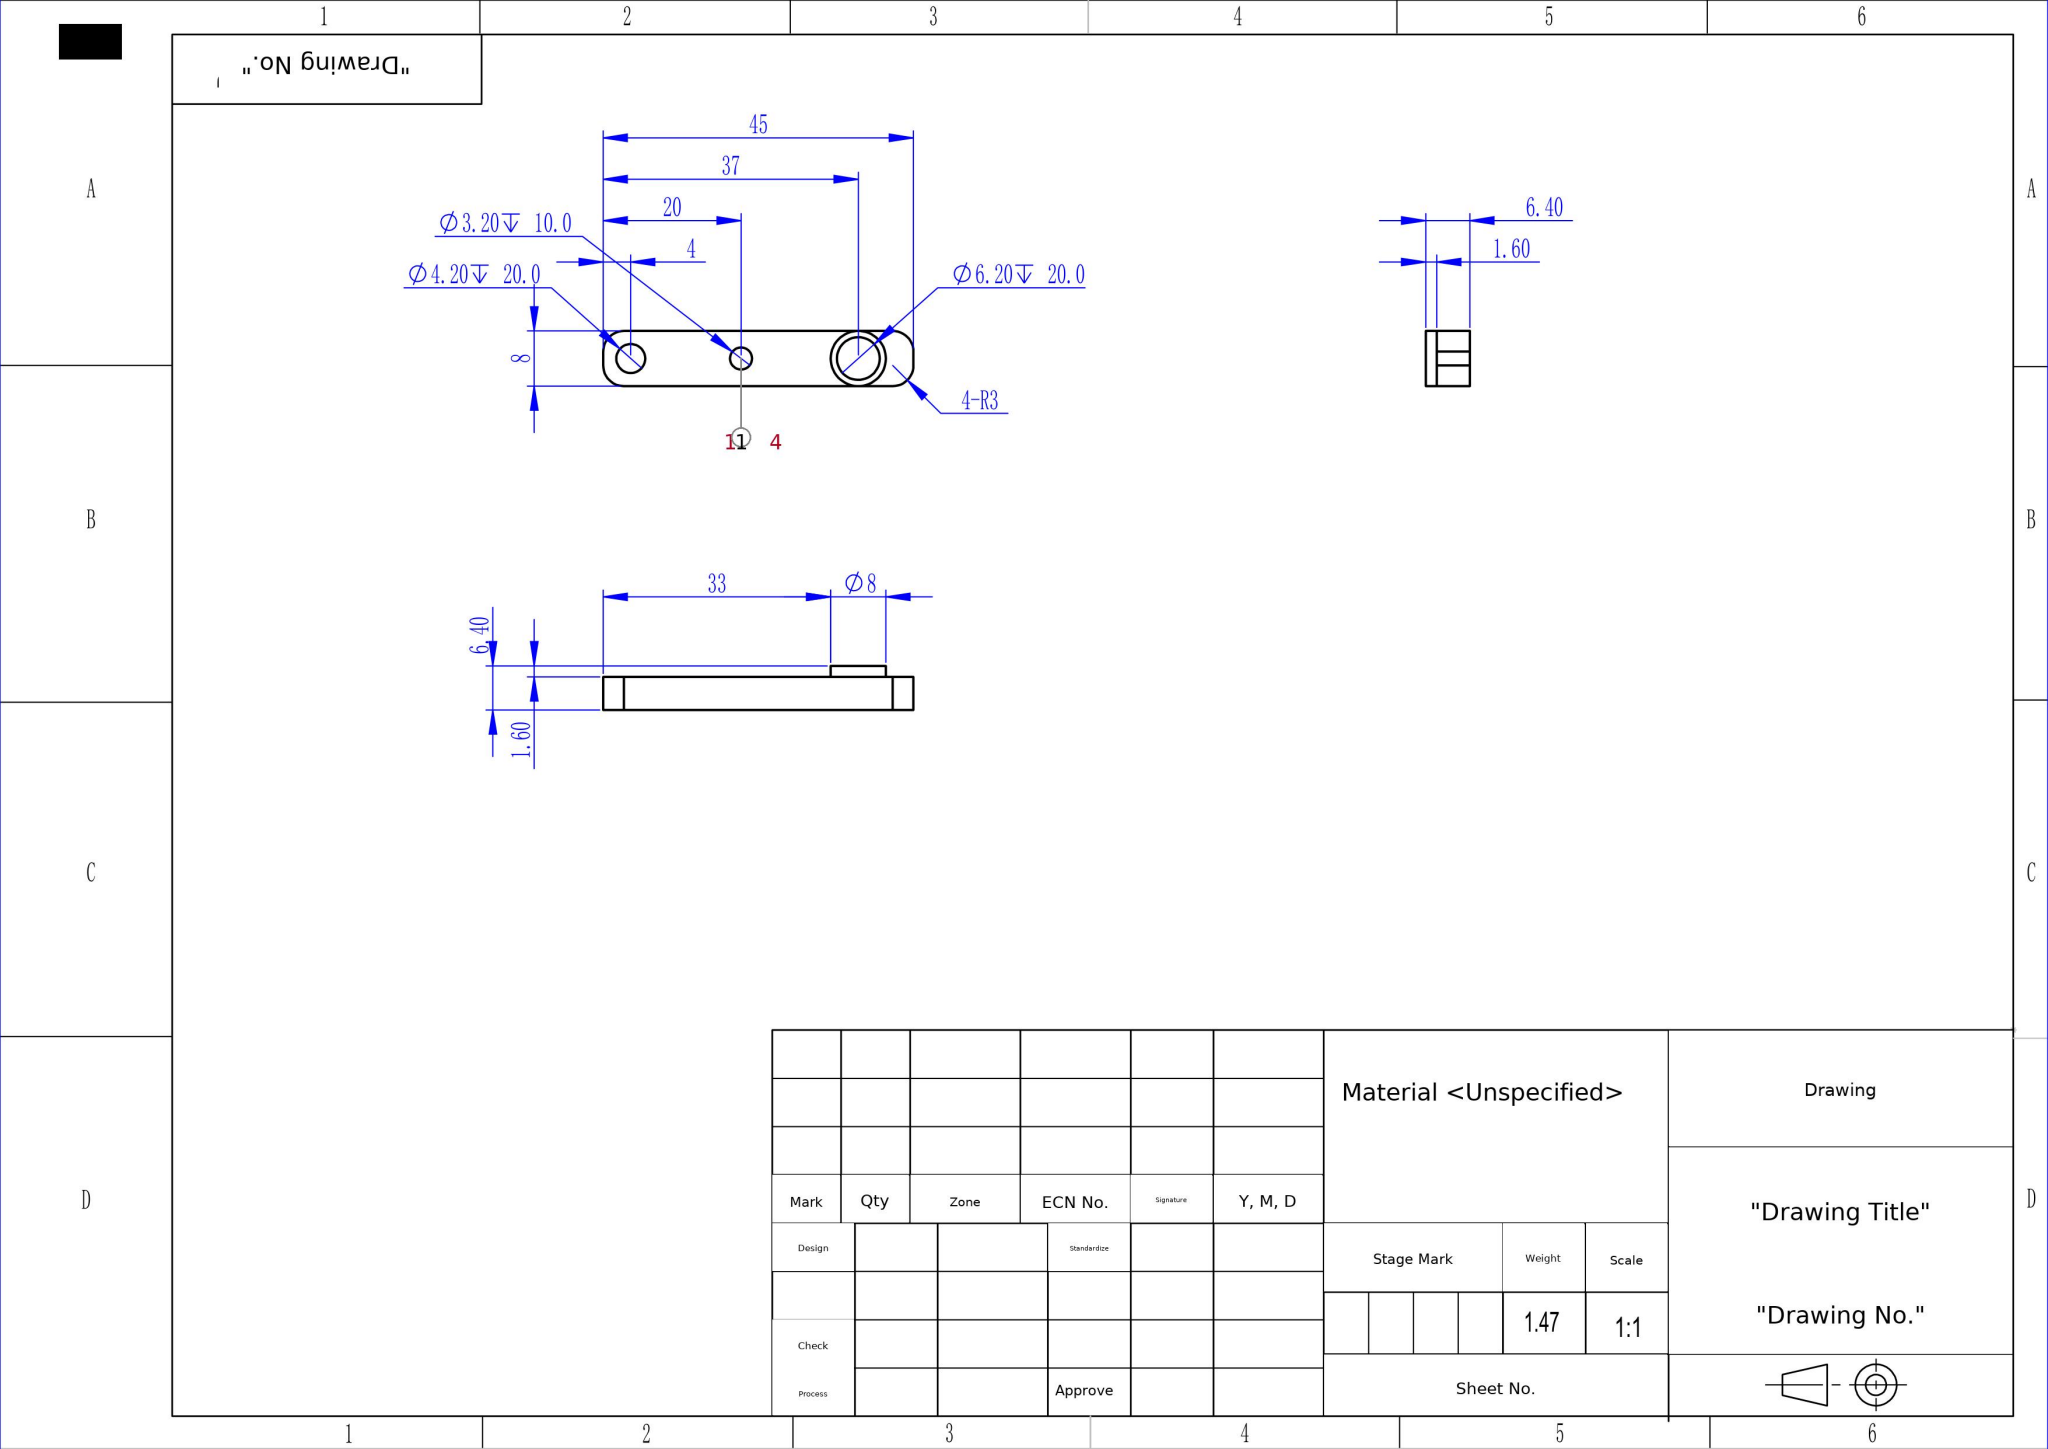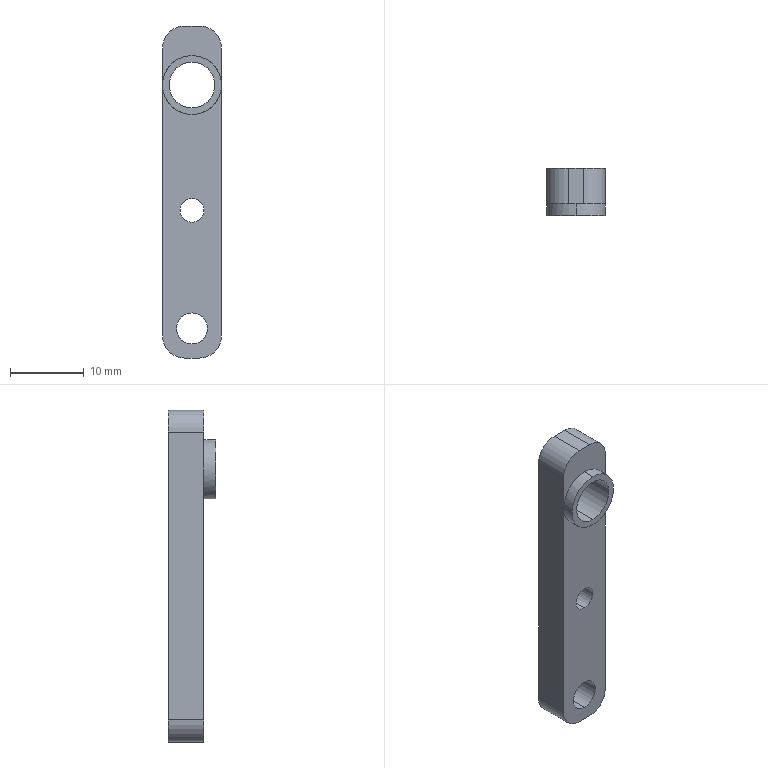Part | SolidWorks | mm | material Unspecified | 1 solid | 20 faces | box 8 x 6.4 x 45 mm | volume 1473 mm3 | cylinder 12 | plane 8 | commonest cylinder face diameters 6 x4 3.2 x2 8 x2 6.2 x2 4.2 x2
build123d program:
from build123d import *

# Parameters (mm, degrees)
SKETCH1_W           = 8
SKETCH1_H           = 4.8
BOSS_EXTRUDE1_DEPTH = 45
SKETCH2_R           = 2.1
CUT_EXTRUDE1_DEPTH  = 20
FILLET1_R           = 3
SKETCH3_R           = 3.1
CUT_EXTRUDE2_DEPTH  = 20
FILLET2_R           = 3
SKETCH4_R           = 4
SKETCH4_R_2         = 3.1
BOSS_EXTRUDE2_DEPTH = 1.6
SKETCH5_R           = 1.6
CUT_EXTRUDE3_DEPTH  = 10


with BuildPart() as part:
    # Sketch1 → Boss-Extrude1 (new body)
    with BuildSketch(Plane.XY):
        Rectangle(SKETCH1_W, SKETCH1_H)
    extrude(amount=BOSS_EXTRUDE1_DEPTH)

    # Sketch2 → Cut-Extrude1 (cut)
    with BuildSketch(Plane(origin=(0, 2.4, 0), x_dir=(1, 0, 0), z_dir=(0, 1, 0))):
        with Locations(Location((0, -4, 0), (0, 0, 270))):
            Circle(SKETCH2_R)
    extrude(amount=-CUT_EXTRUDE1_DEPTH, mode=Mode.SUBTRACT)

    # Fillet1
    fillet1_edges = [part.edges().sort_by_distance(p)[0] for p in [
        (-4, 0, 0),
        (4, 0, 0),
    ]]
    fillet(fillet1_edges, radius=FILLET1_R)

    # Sketch3 → Cut-Extrude2 (cut)
    with BuildSketch(Plane(origin=(0, 2.4, 0), x_dir=(1, 0, 0), z_dir=(0, 1, 0))):
        with Locations(Location((0, -37, 0), (0, 0, 270))):
            Circle(SKETCH3_R)
    extrude(amount=-CUT_EXTRUDE2_DEPTH, mode=Mode.SUBTRACT)

    # Fillet2
    fillet2_edges = [part.edges().sort_by_distance(p)[0] for p in [
        (-4, 0, 45),
        (4, 0, 45),
    ]]
    fillet(fillet2_edges, radius=FILLET2_R)

    # Sketch4 → Boss-Extrude2 (add)
    with BuildSketch(Plane.XZ.offset(2.4)):
        with Locations(Location((0, 37, 0), (0, 0, 90))):
            Circle(SKETCH4_R)
        with Locations(Location((0, 37, 0), (0, 0, 90))):
            Circle(SKETCH4_R_2, mode=Mode.SUBTRACT)
    extrude(amount=BOSS_EXTRUDE2_DEPTH)

    # Sketch5 → Cut-Extrude3 (cut)
    with BuildSketch(Plane(origin=(0, 2.4, 0), x_dir=(1, 0, 0), z_dir=(0, 1, 0))):
        with Locations(Location((0, -20, 0), (0, 0, 270))):
            Circle(SKETCH5_R)
    extrude(amount=-CUT_EXTRUDE3_DEPTH, mode=Mode.SUBTRACT)


solid = part.part
STEP:
#1=CARTESIAN_POINT('',(0.,-2.4,18.4));
#2=VERTEX_POINT('',#1);
#3=CARTESIAN_POINT('',(0.,-2.4,21.6));
#4=VERTEX_POINT('',#3);
#5=CARTESIAN_POINT('',(0.,-2.4,20.));
#6=DIRECTION('',(0.,1.,0.));
#7=DIRECTION('',(0.,0.,1.));
#8=AXIS2_PLACEMENT_3D('',#5,#6,#7);
#9=CIRCLE('',#8,1.6);
#10=EDGE_CURVE('',#2,#4,#9,.T.);
#11=ORIENTED_EDGE('',*,*,#10,.F.);
#12=CARTESIAN_POINT('',(0.,2.4,18.4));
#13=VERTEX_POINT('',#12);
#14=CARTESIAN_POINT('',(0.,-7.6,18.4));
#15=DIRECTION('',(0.,1.,0.));
#16=VECTOR('',#15,1000.);
#17=LINE('',#14,#16);
#18=EDGE_CURVE('',#2,#13,#17,.T.);
#19=ORIENTED_EDGE('',*,*,#18,.T.);
#20=CARTESIAN_POINT('',(0.,2.4,21.6));
#21=VERTEX_POINT('',#20);
#22=CARTESIAN_POINT('',(0.,2.4,20.));
#23=DIRECTION('',(0.,1.,0.));
#24=DIRECTION('',(0.,0.,1.));
#25=AXIS2_PLACEMENT_3D('',#22,#23,#24);
#26=CIRCLE('',#25,1.6);
#27=EDGE_CURVE('',#13,#21,#26,.T.);
#28=ORIENTED_EDGE('',*,*,#27,.T.);
#29=CARTESIAN_POINT('',(0.,-7.6,21.6));
#30=DIRECTION('',(0.,1.,0.));
#31=VECTOR('',#30,1000.);
#32=LINE('',#29,#31);
#33=EDGE_CURVE('',#4,#21,#32,.T.);
#34=ORIENTED_EDGE('',*,*,#33,.F.);
#35=EDGE_LOOP('',(#11,#19,#28,#34));
#36=FACE_OUTER_BOUND('',#35,.T.);
#37=CARTESIAN_POINT('',(0.,-7.6,20.));
#38=DIRECTION('',(0.,1.,0.));
#39=DIRECTION('',(0.,0.,1.));
#40=AXIS2_PLACEMENT_3D('',#37,#38,#39);
#41=CYLINDRICAL_SURFACE('',#40,1.6);
#42=ADVANCED_FACE('',(#36),#41,.F.);
#43=CARTESIAN_POINT('',(0.,-4.,41.));
#44=VERTEX_POINT('',#43);
#45=CARTESIAN_POINT('',(0.,-4.,33.));
#46=VERTEX_POINT('',#45);
#47=CARTESIAN_POINT('',(0.,-4.,37.));
#48=DIRECTION('',(0.,1.,-0.));
#49=DIRECTION('',(0.,0.,1.));
#50=AXIS2_PLACEMENT_3D('',#47,#48,#49);
#51=CIRCLE('',#50,4.);
#52=EDGE_CURVE('',#44,#46,#51,.T.);
#53=ORIENTED_EDGE('',*,*,#52,.T.);
#54=CARTESIAN_POINT('',(0.,-2.4,33.));
#55=VERTEX_POINT('',#54);
#56=CARTESIAN_POINT('',(0.,-15.314,33.));
#57=DIRECTION('',(0.,1.,0.));
#58=VECTOR('',#57,1000.);
#59=LINE('',#56,#58);
#60=EDGE_CURVE('',#46,#55,#59,.T.);
#61=ORIENTED_EDGE('',*,*,#60,.T.);
#62=CARTESIAN_POINT('',(4.,-2.4,37.));
#63=VERTEX_POINT('',#62);
#64=CARTESIAN_POINT('',(0.,-2.4,37.));
#65=DIRECTION('',(0.,-1.,0.));
#66=DIRECTION('',(0.,0.,-1.));
#67=AXIS2_PLACEMENT_3D('',#64,#65,#66);
#68=CIRCLE('',#67,4.);
#69=EDGE_CURVE('',#55,#63,#68,.T.);
#70=ORIENTED_EDGE('',*,*,#69,.T.);
#71=CARTESIAN_POINT('',(0.,-2.4,41.));
#72=VERTEX_POINT('',#71);
#73=CARTESIAN_POINT('',(0.,-2.4,37.));
#74=DIRECTION('',(0.,-1.,0.));
#75=DIRECTION('',(0.,0.,-1.));
#76=AXIS2_PLACEMENT_3D('',#73,#74,#75);
#77=CIRCLE('',#76,4.);
#78=EDGE_CURVE('',#63,#72,#77,.T.);
#79=ORIENTED_EDGE('',*,*,#78,.T.);
#80=CARTESIAN_POINT('',(0.,-15.314,41.));
#81=DIRECTION('',(0.,1.,0.));
#82=VECTOR('',#81,1000.);
#83=LINE('',#80,#82);
#84=EDGE_CURVE('',#44,#72,#83,.T.);
#85=ORIENTED_EDGE('',*,*,#84,.F.);
#86=EDGE_LOOP('',(#53,#61,#70,#79,#85));
#87=FACE_OUTER_BOUND('',#86,.T.);
#88=CARTESIAN_POINT('',(0.,-15.314,37.));
#89=DIRECTION('',(0.,1.,0.));
#90=DIRECTION('',(0.,0.,1.));
#91=AXIS2_PLACEMENT_3D('',#88,#89,#90);
#92=CYLINDRICAL_SURFACE('',#91,4.);
#93=ADVANCED_FACE('',(#87),#92,.T.);
#94=CARTESIAN_POINT('',(0.,-4.,33.9));
#95=VERTEX_POINT('',#94);
#96=CARTESIAN_POINT('',(0.,-4.,40.1));
#97=VERTEX_POINT('',#96);
#98=CARTESIAN_POINT('',(0.,-4.,37.));
#99=DIRECTION('',(0.,1.,-0.));
#100=DIRECTION('',(0.,0.,1.));
#101=AXIS2_PLACEMENT_3D('',#98,#99,#100);
#102=CIRCLE('',#101,3.1);
#103=EDGE_CURVE('',#95,#97,#102,.T.);
#104=ORIENTED_EDGE('',*,*,#103,.F.);
#105=CARTESIAN_POINT('',(0.,2.4,33.9));
#106=VERTEX_POINT('',#105);
#107=CARTESIAN_POINT('',(0.,-17.6,33.9));
#108=DIRECTION('',(0.,1.,0.));
#109=VECTOR('',#108,1000.);
#110=LINE('',#107,#109);
#111=EDGE_CURVE('',#95,#106,#110,.T.);
#112=ORIENTED_EDGE('',*,*,#111,.T.);
#113=CARTESIAN_POINT('',(0.,2.4,40.1));
#114=VERTEX_POINT('',#113);
#115=CARTESIAN_POINT('',(0.,2.4,37.));
#116=DIRECTION('',(0.,1.,0.));
#117=DIRECTION('',(0.,0.,1.));
#118=AXIS2_PLACEMENT_3D('',#115,#116,#117);
#119=CIRCLE('',#118,3.1);
#120=EDGE_CURVE('',#106,#114,#119,.T.);
#121=ORIENTED_EDGE('',*,*,#120,.T.);
#122=CARTESIAN_POINT('',(0.,-17.6,40.1));
#123=DIRECTION('',(0.,1.,0.));
#124=VECTOR('',#123,1000.);
#125=LINE('',#122,#124);
#126=EDGE_CURVE('',#97,#114,#125,.T.);
#127=ORIENTED_EDGE('',*,*,#126,.F.);
#128=EDGE_LOOP('',(#104,#112,#121,#127));
#129=FACE_OUTER_BOUND('',#128,.T.);
#130=CARTESIAN_POINT('',(0.,-17.6,37.));
#131=DIRECTION('',(0.,1.,0.));
#132=DIRECTION('',(0.,0.,1.));
#133=AXIS2_PLACEMENT_3D('',#130,#131,#132);
#134=CYLINDRICAL_SURFACE('',#133,3.1);
#135=ADVANCED_FACE('',(#129),#134,.F.);
#136=CARTESIAN_POINT('',(0.,-2.4,1.9));
#137=VERTEX_POINT('',#136);
#138=CARTESIAN_POINT('',(0.,-2.4,6.1));
#139=VERTEX_POINT('',#138);
#140=CARTESIAN_POINT('',(0.,-2.4,4.));
#141=DIRECTION('',(0.,1.,0.));
#142=DIRECTION('',(0.,0.,1.));
#143=AXIS2_PLACEMENT_3D('',#140,#141,#142);
#144=CIRCLE('',#143,2.1);
#145=EDGE_CURVE('',#137,#139,#144,.T.);
#146=ORIENTED_EDGE('',*,*,#145,.F.);
#147=CARTESIAN_POINT('',(0.,2.4,1.9));
#148=VERTEX_POINT('',#147);
#149=CARTESIAN_POINT('',(0.,-17.6,1.9));
#150=DIRECTION('',(0.,1.,0.));
#151=VECTOR('',#150,1000.);
#152=LINE('',#149,#151);
#153=EDGE_CURVE('',#137,#148,#152,.T.);
#154=ORIENTED_EDGE('',*,*,#153,.T.);
#155=CARTESIAN_POINT('',(0.,2.4,6.1));
#156=VERTEX_POINT('',#155);
#157=CARTESIAN_POINT('',(0.,2.4,4.));
#158=DIRECTION('',(0.,1.,0.));
#159=DIRECTION('',(0.,0.,1.));
#160=AXIS2_PLACEMENT_3D('',#157,#158,#159);
#161=CIRCLE('',#160,2.1);
#162=EDGE_CURVE('',#148,#156,#161,.T.);
#163=ORIENTED_EDGE('',*,*,#162,.T.);
#164=CARTESIAN_POINT('',(0.,-17.6,6.1));
#165=DIRECTION('',(0.,1.,0.));
#166=VECTOR('',#165,1000.);
#167=LINE('',#164,#166);
#168=EDGE_CURVE('',#139,#156,#167,.T.);
#169=ORIENTED_EDGE('',*,*,#168,.F.);
#170=EDGE_LOOP('',(#146,#154,#163,#169));
#171=FACE_OUTER_BOUND('',#170,.T.);
#172=CARTESIAN_POINT('',(0.,-17.6,4.));
#173=DIRECTION('',(0.,1.,0.));
#174=DIRECTION('',(0.,0.,1.));
#175=AXIS2_PLACEMENT_3D('',#172,#173,#174);
#176=CYLINDRICAL_SURFACE('',#175,2.1);
#177=ADVANCED_FACE('',(#171),#176,.F.);
#178=ORIENTED_EDGE('',*,*,#78,.F.);
#179=CARTESIAN_POINT('',(4.,-2.4,42.));
#180=VERTEX_POINT('',#179);
#181=CARTESIAN_POINT('',(4.,-2.4,45.));
#182=DIRECTION('',(0.,0.,-1.));
#183=VECTOR('',#182,1000.);
#184=LINE('',#181,#183);
#185=EDGE_CURVE('',#180,#63,#184,.T.);
#186=ORIENTED_EDGE('',*,*,#185,.F.);
#187=CARTESIAN_POINT('',(1.,-2.4,45.));
#188=VERTEX_POINT('',#187);
#189=CARTESIAN_POINT('',(1.,-2.4,42.));
#190=DIRECTION('',(0.,-1.,0.));
#191=DIRECTION('',(0.,0.,1.));
#192=AXIS2_PLACEMENT_3D('',#189,#190,#191);
#193=CIRCLE('',#192,3.);
#194=EDGE_CURVE('',#180,#188,#193,.T.);
#195=ORIENTED_EDGE('',*,*,#194,.T.);
#196=CARTESIAN_POINT('',(-1.,-2.4,45.));
#197=VERTEX_POINT('',#196);
#198=CARTESIAN_POINT('',(-4.,-2.4,45.));
#199=DIRECTION('',(1.,0.,0.));
#200=VECTOR('',#199,1000.);
#201=LINE('',#198,#200);
#202=EDGE_CURVE('',#197,#188,#201,.T.);
#203=ORIENTED_EDGE('',*,*,#202,.F.);
#204=CARTESIAN_POINT('',(-4.,-2.4,42.));
#205=VERTEX_POINT('',#204);
#206=CARTESIAN_POINT('',(-1.,-2.4,42.));
#207=DIRECTION('',(0.,-1.,0.));
#208=DIRECTION('',(0.,0.,1.));
#209=AXIS2_PLACEMENT_3D('',#206,#207,#208);
#210=CIRCLE('',#209,3.);
#211=EDGE_CURVE('',#197,#205,#210,.T.);
#212=ORIENTED_EDGE('',*,*,#211,.T.);
#213=CARTESIAN_POINT('',(-4.,-2.4,37.));
#214=VERTEX_POINT('',#213);
#215=CARTESIAN_POINT('',(-4.,-2.4,45.));
#216=DIRECTION('',(0.,0.,-1.));
#217=VECTOR('',#216,1000.);
#218=LINE('',#215,#217);
#219=EDGE_CURVE('',#205,#214,#218,.T.);
#220=ORIENTED_EDGE('',*,*,#219,.T.);
#221=CARTESIAN_POINT('',(0.,-2.4,37.));
#222=DIRECTION('',(0.,-1.,0.));
#223=DIRECTION('',(0.,0.,-1.));
#224=AXIS2_PLACEMENT_3D('',#221,#222,#223);
#225=CIRCLE('',#224,4.);
#226=EDGE_CURVE('',#72,#214,#225,.T.);
#227=ORIENTED_EDGE('',*,*,#226,.F.);
#228=EDGE_LOOP('',(#178,#186,#195,#203,#212,#220,#227));
#229=FACE_OUTER_BOUND('',#228,.T.);
#230=CARTESIAN_POINT('',(-4.,-2.4,45.));
#231=DIRECTION('',(0.,1.,0.));
#232=DIRECTION('',(0.,0.,1.));
#233=AXIS2_PLACEMENT_3D('',#230,#231,#232);
#234=PLANE('',#233);
#235=ADVANCED_FACE('',(#229),#234,.F.);
#236=CARTESIAN_POINT('',(4.,2.4,42.));
#237=VERTEX_POINT('',#236);
#238=CARTESIAN_POINT('',(4.,2.4,3.));
#239=VERTEX_POINT('',#238);
#240=CARTESIAN_POINT('',(4.,2.4,45.));
#241=DIRECTION('',(0.,0.,-1.));
#242=VECTOR('',#241,1000.);
#243=LINE('',#240,#242);
#244=EDGE_CURVE('',#237,#239,#243,.T.);
#245=ORIENTED_EDGE('',*,*,#244,.F.);
#246=CARTESIAN_POINT('',(4.,-2.4,42.));
#247=DIRECTION('',(0.,-1.,0.));
#248=VECTOR('',#247,1000.);
#249=LINE('',#246,#248);
#250=EDGE_CURVE('',#237,#180,#249,.T.);
#251=ORIENTED_EDGE('',*,*,#250,.T.);
#252=ORIENTED_EDGE('',*,*,#185,.T.);
#253=CARTESIAN_POINT('',(4.,-2.4,3.));
#254=VERTEX_POINT('',#253);
#255=CARTESIAN_POINT('',(4.,-2.4,45.));
#256=DIRECTION('',(0.,0.,-1.));
#257=VECTOR('',#256,1000.);
#258=LINE('',#255,#257);
#259=EDGE_CURVE('',#63,#254,#258,.T.);
#260=ORIENTED_EDGE('',*,*,#259,.T.);
#261=CARTESIAN_POINT('',(4.,2.4,3.));
#262=DIRECTION('',(-0.,1.,0.));
#263=VECTOR('',#262,1000.);
#264=LINE('',#261,#263);
#265=EDGE_CURVE('',#254,#239,#264,.T.);
#266=ORIENTED_EDGE('',*,*,#265,.T.);
#267=EDGE_LOOP('',(#245,#251,#252,#260,#266));
#268=FACE_OUTER_BOUND('',#267,.T.);
#269=CARTESIAN_POINT('',(4.,2.4,45.));
#270=DIRECTION('',(-1.,-0.,0.));
#271=DIRECTION('',(0.,-1.,0.));
#272=AXIS2_PLACEMENT_3D('',#269,#270,#271);
#273=PLANE('',#272);
#274=ADVANCED_FACE('',(#268),#273,.F.);
#275=CARTESIAN_POINT('',(0.,2.4,20.));
#276=DIRECTION('',(0.,1.,0.));
#277=DIRECTION('',(0.,0.,1.));
#278=AXIS2_PLACEMENT_3D('',#275,#276,#277);
#279=CIRCLE('',#278,1.6);
#280=EDGE_CURVE('',#21,#13,#279,.T.);
#281=ORIENTED_EDGE('',*,*,#280,.F.);
#282=ORIENTED_EDGE('',*,*,#27,.F.);
#283=EDGE_LOOP('',(#281,#282));
#284=FACE_BOUND('',#283,.T.);
#285=CARTESIAN_POINT('',(0.,2.4,37.));
#286=DIRECTION('',(0.,1.,0.));
#287=DIRECTION('',(0.,0.,1.));
#288=AXIS2_PLACEMENT_3D('',#285,#286,#287);
#289=CIRCLE('',#288,3.1);
#290=EDGE_CURVE('',#114,#106,#289,.T.);
#291=ORIENTED_EDGE('',*,*,#290,.F.);
#292=ORIENTED_EDGE('',*,*,#120,.F.);
#293=EDGE_LOOP('',(#291,#292));
#294=FACE_BOUND('',#293,.T.);
#295=CARTESIAN_POINT('',(0.,2.4,4.));
#296=DIRECTION('',(0.,1.,0.));
#297=DIRECTION('',(0.,0.,1.));
#298=AXIS2_PLACEMENT_3D('',#295,#296,#297);
#299=CIRCLE('',#298,2.1);
#300=EDGE_CURVE('',#156,#148,#299,.T.);
#301=ORIENTED_EDGE('',*,*,#300,.F.);
#302=ORIENTED_EDGE('',*,*,#162,.F.);
#303=EDGE_LOOP('',(#301,#302));
#304=FACE_BOUND('',#303,.T.);
#305=CARTESIAN_POINT('',(-4.,2.4,42.));
#306=VERTEX_POINT('',#305);
#307=CARTESIAN_POINT('',(-4.,2.4,3.));
#308=VERTEX_POINT('',#307);
#309=CARTESIAN_POINT('',(-4.,2.4,45.));
#310=DIRECTION('',(0.,0.,-1.));
#311=VECTOR('',#310,1000.);
#312=LINE('',#309,#311);
#313=EDGE_CURVE('',#306,#308,#312,.T.);
#314=ORIENTED_EDGE('',*,*,#313,.F.);
#315=CARTESIAN_POINT('',(-1.,2.4,45.));
#316=VERTEX_POINT('',#315);
#317=CARTESIAN_POINT('',(-1.,2.4,42.));
#318=DIRECTION('',(0.,1.,0.));
#319=DIRECTION('',(0.,0.,-1.));
#320=AXIS2_PLACEMENT_3D('',#317,#318,#319);
#321=CIRCLE('',#320,3.);
#322=EDGE_CURVE('',#306,#316,#321,.T.);
#323=ORIENTED_EDGE('',*,*,#322,.T.);
#324=CARTESIAN_POINT('',(1.,2.4,45.));
#325=VERTEX_POINT('',#324);
#326=CARTESIAN_POINT('',(-4.,2.4,45.));
#327=DIRECTION('',(-1.,0.,0.));
#328=VECTOR('',#327,1000.);
#329=LINE('',#326,#328);
#330=EDGE_CURVE('',#325,#316,#329,.T.);
#331=ORIENTED_EDGE('',*,*,#330,.F.);
#332=CARTESIAN_POINT('',(1.,2.4,42.));
#333=DIRECTION('',(0.,1.,0.));
#334=DIRECTION('',(0.,0.,-1.));
#335=AXIS2_PLACEMENT_3D('',#332,#333,#334);
#336=CIRCLE('',#335,3.);
#337=EDGE_CURVE('',#325,#237,#336,.T.);
#338=ORIENTED_EDGE('',*,*,#337,.T.);
#339=ORIENTED_EDGE('',*,*,#244,.T.);
#340=CARTESIAN_POINT('',(1.,2.4,0.));
#341=VERTEX_POINT('',#340);
#342=CARTESIAN_POINT('',(1.,2.4,3.));
#343=DIRECTION('',(0.,1.,0.));
#344=DIRECTION('',(0.,0.,-1.));
#345=AXIS2_PLACEMENT_3D('',#342,#343,#344);
#346=CIRCLE('',#345,3.);
#347=EDGE_CURVE('',#239,#341,#346,.T.);
#348=ORIENTED_EDGE('',*,*,#347,.T.);
#349=CARTESIAN_POINT('',(-1.,2.4,0.));
#350=VERTEX_POINT('',#349);
#351=CARTESIAN_POINT('',(-4.,2.4,0.));
#352=DIRECTION('',(-1.,0.,0.));
#353=VECTOR('',#352,1000.);
#354=LINE('',#351,#353);
#355=EDGE_CURVE('',#341,#350,#354,.T.);
#356=ORIENTED_EDGE('',*,*,#355,.T.);
#357=CARTESIAN_POINT('',(-1.,2.4,3.));
#358=DIRECTION('',(0.,1.,0.));
#359=DIRECTION('',(0.,0.,-1.));
#360=AXIS2_PLACEMENT_3D('',#357,#358,#359);
#361=CIRCLE('',#360,3.);
#362=EDGE_CURVE('',#350,#308,#361,.T.);
#363=ORIENTED_EDGE('',*,*,#362,.T.);
#364=EDGE_LOOP('',(#314,#323,#331,#338,#339,#348,#356,#363));
#365=FACE_OUTER_BOUND('',#364,.T.);
#366=CARTESIAN_POINT('',(-4.,2.4,45.));
#367=DIRECTION('',(0.,-1.,0.));
#368=DIRECTION('',(0.,0.,-1.));
#369=AXIS2_PLACEMENT_3D('',#366,#367,#368);
#370=PLANE('',#369);
#371=ADVANCED_FACE('',(#284,#294,#304,#365),#370,.F.);
#372=ORIENTED_EDGE('',*,*,#219,.F.);
#373=CARTESIAN_POINT('',(-4.,2.4,42.));
#374=DIRECTION('',(-0.,1.,0.));
#375=VECTOR('',#374,1000.);
#376=LINE('',#373,#375);
#377=EDGE_CURVE('',#205,#306,#376,.T.);
#378=ORIENTED_EDGE('',*,*,#377,.T.);
#379=ORIENTED_EDGE('',*,*,#313,.T.);
#380=CARTESIAN_POINT('',(-4.,-2.4,3.));
#381=VERTEX_POINT('',#380);
#382=CARTESIAN_POINT('',(-4.,2.4,3.));
#383=DIRECTION('',(0.,-1.,0.));
#384=VECTOR('',#383,1000.);
#385=LINE('',#382,#384);
#386=EDGE_CURVE('',#308,#381,#385,.T.);
#387=ORIENTED_EDGE('',*,*,#386,.T.);
#388=CARTESIAN_POINT('',(-4.,-2.4,45.));
#389=DIRECTION('',(0.,0.,-1.));
#390=VECTOR('',#389,1000.);
#391=LINE('',#388,#390);
#392=EDGE_CURVE('',#214,#381,#391,.T.);
#393=ORIENTED_EDGE('',*,*,#392,.F.);
#394=EDGE_LOOP('',(#372,#378,#379,#387,#393));
#395=FACE_OUTER_BOUND('',#394,.T.);
#396=CARTESIAN_POINT('',(-4.,2.4,45.));
#397=DIRECTION('',(1.,0.,0.));
#398=DIRECTION('',(-0.,1.,0.));
#399=AXIS2_PLACEMENT_3D('',#396,#397,#398);
#400=PLANE('',#399);
#401=ADVANCED_FACE('',(#395),#400,.F.);
#402=CARTESIAN_POINT('',(0.,-2.4,20.));
#403=DIRECTION('',(0.,1.,0.));
#404=DIRECTION('',(0.,0.,1.));
#405=AXIS2_PLACEMENT_3D('',#402,#403,#404);
#406=CIRCLE('',#405,1.6);
#407=EDGE_CURVE('',#4,#2,#406,.T.);
#408=ORIENTED_EDGE('',*,*,#407,.T.);
#409=ORIENTED_EDGE('',*,*,#10,.T.);
#410=EDGE_LOOP('',(#408,#409));
#411=FACE_BOUND('',#410,.T.);
#412=CARTESIAN_POINT('',(0.,-2.4,37.));
#413=DIRECTION('',(0.,-1.,0.));
#414=DIRECTION('',(0.,0.,-1.));
#415=AXIS2_PLACEMENT_3D('',#412,#413,#414);
#416=CIRCLE('',#415,4.);
#417=EDGE_CURVE('',#214,#55,#416,.T.);
#418=ORIENTED_EDGE('',*,*,#417,.F.);
#419=ORIENTED_EDGE('',*,*,#392,.T.);
#420=CARTESIAN_POINT('',(-1.,-2.4,0.));
#421=VERTEX_POINT('',#420);
#422=CARTESIAN_POINT('',(-1.,-2.4,3.));
#423=DIRECTION('',(0.,-1.,0.));
#424=DIRECTION('',(0.,0.,1.));
#425=AXIS2_PLACEMENT_3D('',#422,#423,#424);
#426=CIRCLE('',#425,3.);
#427=EDGE_CURVE('',#381,#421,#426,.T.);
#428=ORIENTED_EDGE('',*,*,#427,.T.);
#429=CARTESIAN_POINT('',(1.,-2.4,0.));
#430=VERTEX_POINT('',#429);
#431=CARTESIAN_POINT('',(-4.,-2.4,0.));
#432=DIRECTION('',(1.,0.,0.));
#433=VECTOR('',#432,1000.);
#434=LINE('',#431,#433);
#435=EDGE_CURVE('',#421,#430,#434,.T.);
#436=ORIENTED_EDGE('',*,*,#435,.T.);
#437=CARTESIAN_POINT('',(1.,-2.4,3.));
#438=DIRECTION('',(0.,-1.,0.));
#439=DIRECTION('',(0.,0.,1.));
#440=AXIS2_PLACEMENT_3D('',#437,#438,#439);
#441=CIRCLE('',#440,3.);
#442=EDGE_CURVE('',#430,#254,#441,.T.);
#443=ORIENTED_EDGE('',*,*,#442,.T.);
#444=ORIENTED_EDGE('',*,*,#259,.F.);
#445=ORIENTED_EDGE('',*,*,#69,.F.);
#446=EDGE_LOOP('',(#418,#419,#428,#436,#443,#444,#445));
#447=FACE_OUTER_BOUND('',#446,.T.);
#448=CARTESIAN_POINT('',(0.,-2.4,4.));
#449=DIRECTION('',(0.,1.,0.));
#450=DIRECTION('',(0.,0.,1.));
#451=AXIS2_PLACEMENT_3D('',#448,#449,#450);
#452=CIRCLE('',#451,2.1);
#453=EDGE_CURVE('',#139,#137,#452,.T.);
#454=ORIENTED_EDGE('',*,*,#453,.T.);
#455=ORIENTED_EDGE('',*,*,#145,.T.);
#456=EDGE_LOOP('',(#454,#455));
#457=FACE_BOUND('',#456,.T.);
#458=CARTESIAN_POINT('',(-4.,-2.4,45.));
#459=DIRECTION('',(0.,1.,0.));
#460=DIRECTION('',(0.,0.,1.));
#461=AXIS2_PLACEMENT_3D('',#458,#459,#460);
#462=PLANE('',#461);
#463=ADVANCED_FACE('',(#411,#447,#457),#462,.F.);
#464=ORIENTED_EDGE('',*,*,#330,.T.);
#465=CARTESIAN_POINT('',(-1.,-2.4,45.));
#466=DIRECTION('',(0.,-1.,0.));
#467=VECTOR('',#466,1000.);
#468=LINE('',#465,#467);
#469=EDGE_CURVE('',#316,#197,#468,.T.);
#470=ORIENTED_EDGE('',*,*,#469,.T.);
#471=ORIENTED_EDGE('',*,*,#202,.T.);
#472=CARTESIAN_POINT('',(1.,2.4,45.));
#473=DIRECTION('',(-0.,1.,0.));
#474=VECTOR('',#473,1000.);
#475=LINE('',#472,#474);
#476=EDGE_CURVE('',#188,#325,#475,.T.);
#477=ORIENTED_EDGE('',*,*,#476,.T.);
#478=EDGE_LOOP('',(#464,#470,#471,#477));
#479=FACE_OUTER_BOUND('',#478,.T.);
#480=CARTESIAN_POINT('',(0.,0.,45.));
#481=DIRECTION('',(0.,0.,1.));
#482=DIRECTION('',(1.,0.,0.));
#483=AXIS2_PLACEMENT_3D('',#480,#481,#482);
#484=PLANE('',#483);
#485=ADVANCED_FACE('',(#479),#484,.T.);
#486=ORIENTED_EDGE('',*,*,#435,.F.);
#487=CARTESIAN_POINT('',(-1.,-0.,0.));
#488=DIRECTION('',(-0.,1.,0.));
#489=VECTOR('',#488,1000.);
#490=LINE('',#487,#489);
#491=EDGE_CURVE('',#421,#350,#490,.T.);
#492=ORIENTED_EDGE('',*,*,#491,.T.);
#493=ORIENTED_EDGE('',*,*,#355,.F.);
#494=CARTESIAN_POINT('',(1.,0.,0.));
#495=DIRECTION('',(0.,-1.,0.));
#496=VECTOR('',#495,1000.);
#497=LINE('',#494,#496);
#498=EDGE_CURVE('',#341,#430,#497,.T.);
#499=ORIENTED_EDGE('',*,*,#498,.T.);
#500=EDGE_LOOP('',(#486,#492,#493,#499));
#501=FACE_OUTER_BOUND('',#500,.T.);
#502=CARTESIAN_POINT('',(0.,0.,0.));
#503=DIRECTION('',(0.,0.,1.));
#504=DIRECTION('',(1.,0.,0.));
#505=AXIS2_PLACEMENT_3D('',#502,#503,#504);
#506=PLANE('',#505);
#507=ADVANCED_FACE('',(#501),#506,.F.);
#508=ORIENTED_EDGE('',*,*,#153,.F.);
#509=ORIENTED_EDGE('',*,*,#453,.F.);
#510=ORIENTED_EDGE('',*,*,#168,.T.);
#511=ORIENTED_EDGE('',*,*,#300,.T.);
#512=EDGE_LOOP('',(#508,#509,#510,#511));
#513=FACE_OUTER_BOUND('',#512,.T.);
#514=CARTESIAN_POINT('',(0.,-17.6,4.));
#515=DIRECTION('',(0.,1.,0.));
#516=DIRECTION('',(0.,0.,1.));
#517=AXIS2_PLACEMENT_3D('',#514,#515,#516);
#518=CYLINDRICAL_SURFACE('',#517,2.1);
#519=ADVANCED_FACE('',(#513),#518,.F.);
#520=ORIENTED_EDGE('',*,*,#362,.F.);
#521=ORIENTED_EDGE('',*,*,#491,.F.);
#522=ORIENTED_EDGE('',*,*,#427,.F.);
#523=ORIENTED_EDGE('',*,*,#386,.F.);
#524=EDGE_LOOP('',(#520,#521,#522,#523));
#525=FACE_OUTER_BOUND('',#524,.T.);
#526=CARTESIAN_POINT('',(-1.,2.4,3.));
#527=DIRECTION('',(0.,-1.,0.));
#528=DIRECTION('',(1.,0.,0.));
#529=AXIS2_PLACEMENT_3D('',#526,#527,#528);
#530=CYLINDRICAL_SURFACE('',#529,3.);
#531=ADVANCED_FACE('',(#525),#530,.T.);
#532=ORIENTED_EDGE('',*,*,#442,.F.);
#533=ORIENTED_EDGE('',*,*,#498,.F.);
#534=ORIENTED_EDGE('',*,*,#347,.F.);
#535=ORIENTED_EDGE('',*,*,#265,.F.);
#536=EDGE_LOOP('',(#532,#533,#534,#535));
#537=FACE_OUTER_BOUND('',#536,.T.);
#538=CARTESIAN_POINT('',(1.,2.4,3.));
#539=DIRECTION('',(-0.,1.,0.));
#540=DIRECTION('',(-1.,-0.,0.));
#541=AXIS2_PLACEMENT_3D('',#538,#539,#540);
#542=CYLINDRICAL_SURFACE('',#541,3.);
#543=ADVANCED_FACE('',(#537),#542,.T.);
#544=ORIENTED_EDGE('',*,*,#111,.F.);
#545=CARTESIAN_POINT('',(0.,-4.,37.));
#546=DIRECTION('',(0.,1.,-0.));
#547=DIRECTION('',(0.,0.,1.));
#548=AXIS2_PLACEMENT_3D('',#545,#546,#547);
#549=CIRCLE('',#548,3.1);
#550=EDGE_CURVE('',#97,#95,#549,.T.);
#551=ORIENTED_EDGE('',*,*,#550,.F.);
#552=ORIENTED_EDGE('',*,*,#126,.T.);
#553=ORIENTED_EDGE('',*,*,#290,.T.);
#554=EDGE_LOOP('',(#544,#551,#552,#553));
#555=FACE_OUTER_BOUND('',#554,.T.);
#556=CARTESIAN_POINT('',(0.,-17.6,37.));
#557=DIRECTION('',(0.,1.,0.));
#558=DIRECTION('',(0.,0.,1.));
#559=AXIS2_PLACEMENT_3D('',#556,#557,#558);
#560=CYLINDRICAL_SURFACE('',#559,3.1);
#561=ADVANCED_FACE('',(#555),#560,.F.);
#562=ORIENTED_EDGE('',*,*,#322,.F.);
#563=ORIENTED_EDGE('',*,*,#377,.F.);
#564=ORIENTED_EDGE('',*,*,#211,.F.);
#565=ORIENTED_EDGE('',*,*,#469,.F.);
#566=EDGE_LOOP('',(#562,#563,#564,#565));
#567=FACE_OUTER_BOUND('',#566,.T.);
#568=CARTESIAN_POINT('',(-1.,-0.,42.));
#569=DIRECTION('',(-0.,1.,0.));
#570=DIRECTION('',(-1.,-0.,0.));
#571=AXIS2_PLACEMENT_3D('',#568,#569,#570);
#572=CYLINDRICAL_SURFACE('',#571,3.);
#573=ADVANCED_FACE('',(#567),#572,.T.);
#574=ORIENTED_EDGE('',*,*,#194,.F.);
#575=ORIENTED_EDGE('',*,*,#250,.F.);
#576=ORIENTED_EDGE('',*,*,#337,.F.);
#577=ORIENTED_EDGE('',*,*,#476,.F.);
#578=EDGE_LOOP('',(#574,#575,#576,#577));
#579=FACE_OUTER_BOUND('',#578,.T.);
#580=CARTESIAN_POINT('',(1.,0.,42.));
#581=DIRECTION('',(0.,-1.,0.));
#582=DIRECTION('',(1.,0.,0.));
#583=AXIS2_PLACEMENT_3D('',#580,#581,#582);
#584=CYLINDRICAL_SURFACE('',#583,3.);
#585=ADVANCED_FACE('',(#579),#584,.T.);
#586=ORIENTED_EDGE('',*,*,#60,.F.);
#587=CARTESIAN_POINT('',(0.,-4.,37.));
#588=DIRECTION('',(0.,1.,-0.));
#589=DIRECTION('',(0.,0.,1.));
#590=AXIS2_PLACEMENT_3D('',#587,#588,#589);
#591=CIRCLE('',#590,4.);
#592=EDGE_CURVE('',#46,#44,#591,.T.);
#593=ORIENTED_EDGE('',*,*,#592,.T.);
#594=ORIENTED_EDGE('',*,*,#84,.T.);
#595=ORIENTED_EDGE('',*,*,#226,.T.);
#596=ORIENTED_EDGE('',*,*,#417,.T.);
#597=EDGE_LOOP('',(#586,#593,#594,#595,#596));
#598=FACE_OUTER_BOUND('',#597,.T.);
#599=CARTESIAN_POINT('',(0.,-15.314,37.));
#600=DIRECTION('',(0.,1.,0.));
#601=DIRECTION('',(0.,0.,1.));
#602=AXIS2_PLACEMENT_3D('',#599,#600,#601);
#603=CYLINDRICAL_SURFACE('',#602,4.);
#604=ADVANCED_FACE('',(#598),#603,.T.);
#605=ORIENTED_EDGE('',*,*,#550,.T.);
#606=ORIENTED_EDGE('',*,*,#103,.T.);
#607=EDGE_LOOP('',(#605,#606));
#608=FACE_BOUND('',#607,.T.);
#609=ORIENTED_EDGE('',*,*,#52,.F.);
#610=ORIENTED_EDGE('',*,*,#592,.F.);
#611=EDGE_LOOP('',(#609,#610));
#612=FACE_OUTER_BOUND('',#611,.T.);
#613=CARTESIAN_POINT('',(0.,-4.,37.));
#614=DIRECTION('',(0.,1.,-0.));
#615=DIRECTION('',(0.,-0.,-1.));
#616=AXIS2_PLACEMENT_3D('',#613,#614,#615);
#617=PLANE('',#616);
#618=ADVANCED_FACE('',(#608,#612),#617,.F.);
#619=ORIENTED_EDGE('',*,*,#18,.F.);
#620=ORIENTED_EDGE('',*,*,#407,.F.);
#621=ORIENTED_EDGE('',*,*,#33,.T.);
#622=ORIENTED_EDGE('',*,*,#280,.T.);
#623=EDGE_LOOP('',(#619,#620,#621,#622));
#624=FACE_OUTER_BOUND('',#623,.T.);
#625=CARTESIAN_POINT('',(0.,-7.6,20.));
#626=DIRECTION('',(0.,1.,0.));
#627=DIRECTION('',(0.,0.,1.));
#628=AXIS2_PLACEMENT_3D('',#625,#626,#627);
#629=CYLINDRICAL_SURFACE('',#628,1.6);
#630=ADVANCED_FACE('',(#624),#629,.F.);
#631=CLOSED_SHELL('',(#42,#93,#135,#177,#235,#274,#371,#401,#463,#485,#507,#519,#531,#543,#561,#573,#585,#604,#618,#630));
#632=MANIFOLD_SOLID_BREP('',#631);
#633=CARTESIAN_POINT('',(0.,0.,0.));
#634=DIRECTION('',(0.,0.,1.));
#635=DIRECTION('',(1.,0.,0.));
#636=AXIS2_PLACEMENT_3D('',#633,#634,#635);
#637=(LENGTH_UNIT()NAMED_UNIT(*)SI_UNIT(.MILLI.,.METRE.));
#638=UNCERTAINTY_MEASURE_WITH_UNIT(LENGTH_MEASURE(0.00001),#637,'','');
#639=(NAMED_UNIT(*)PLANE_ANGLE_UNIT()SI_UNIT($,.RADIAN.));
#640=(NAMED_UNIT(*)SI_UNIT($,.STERADIAN.)SOLID_ANGLE_UNIT());
#641=(GEOMETRIC_REPRESENTATION_CONTEXT(3)GLOBAL_UNCERTAINTY_ASSIGNED_CONTEXT((#638))GLOBAL_UNIT_ASSIGNED_CONTEXT((#637,#639,#640))REPRESENTATION_CONTEXT('',''));
#642=ADVANCED_BREP_SHAPE_REPRESENTATION('',(#632,#636),#641);